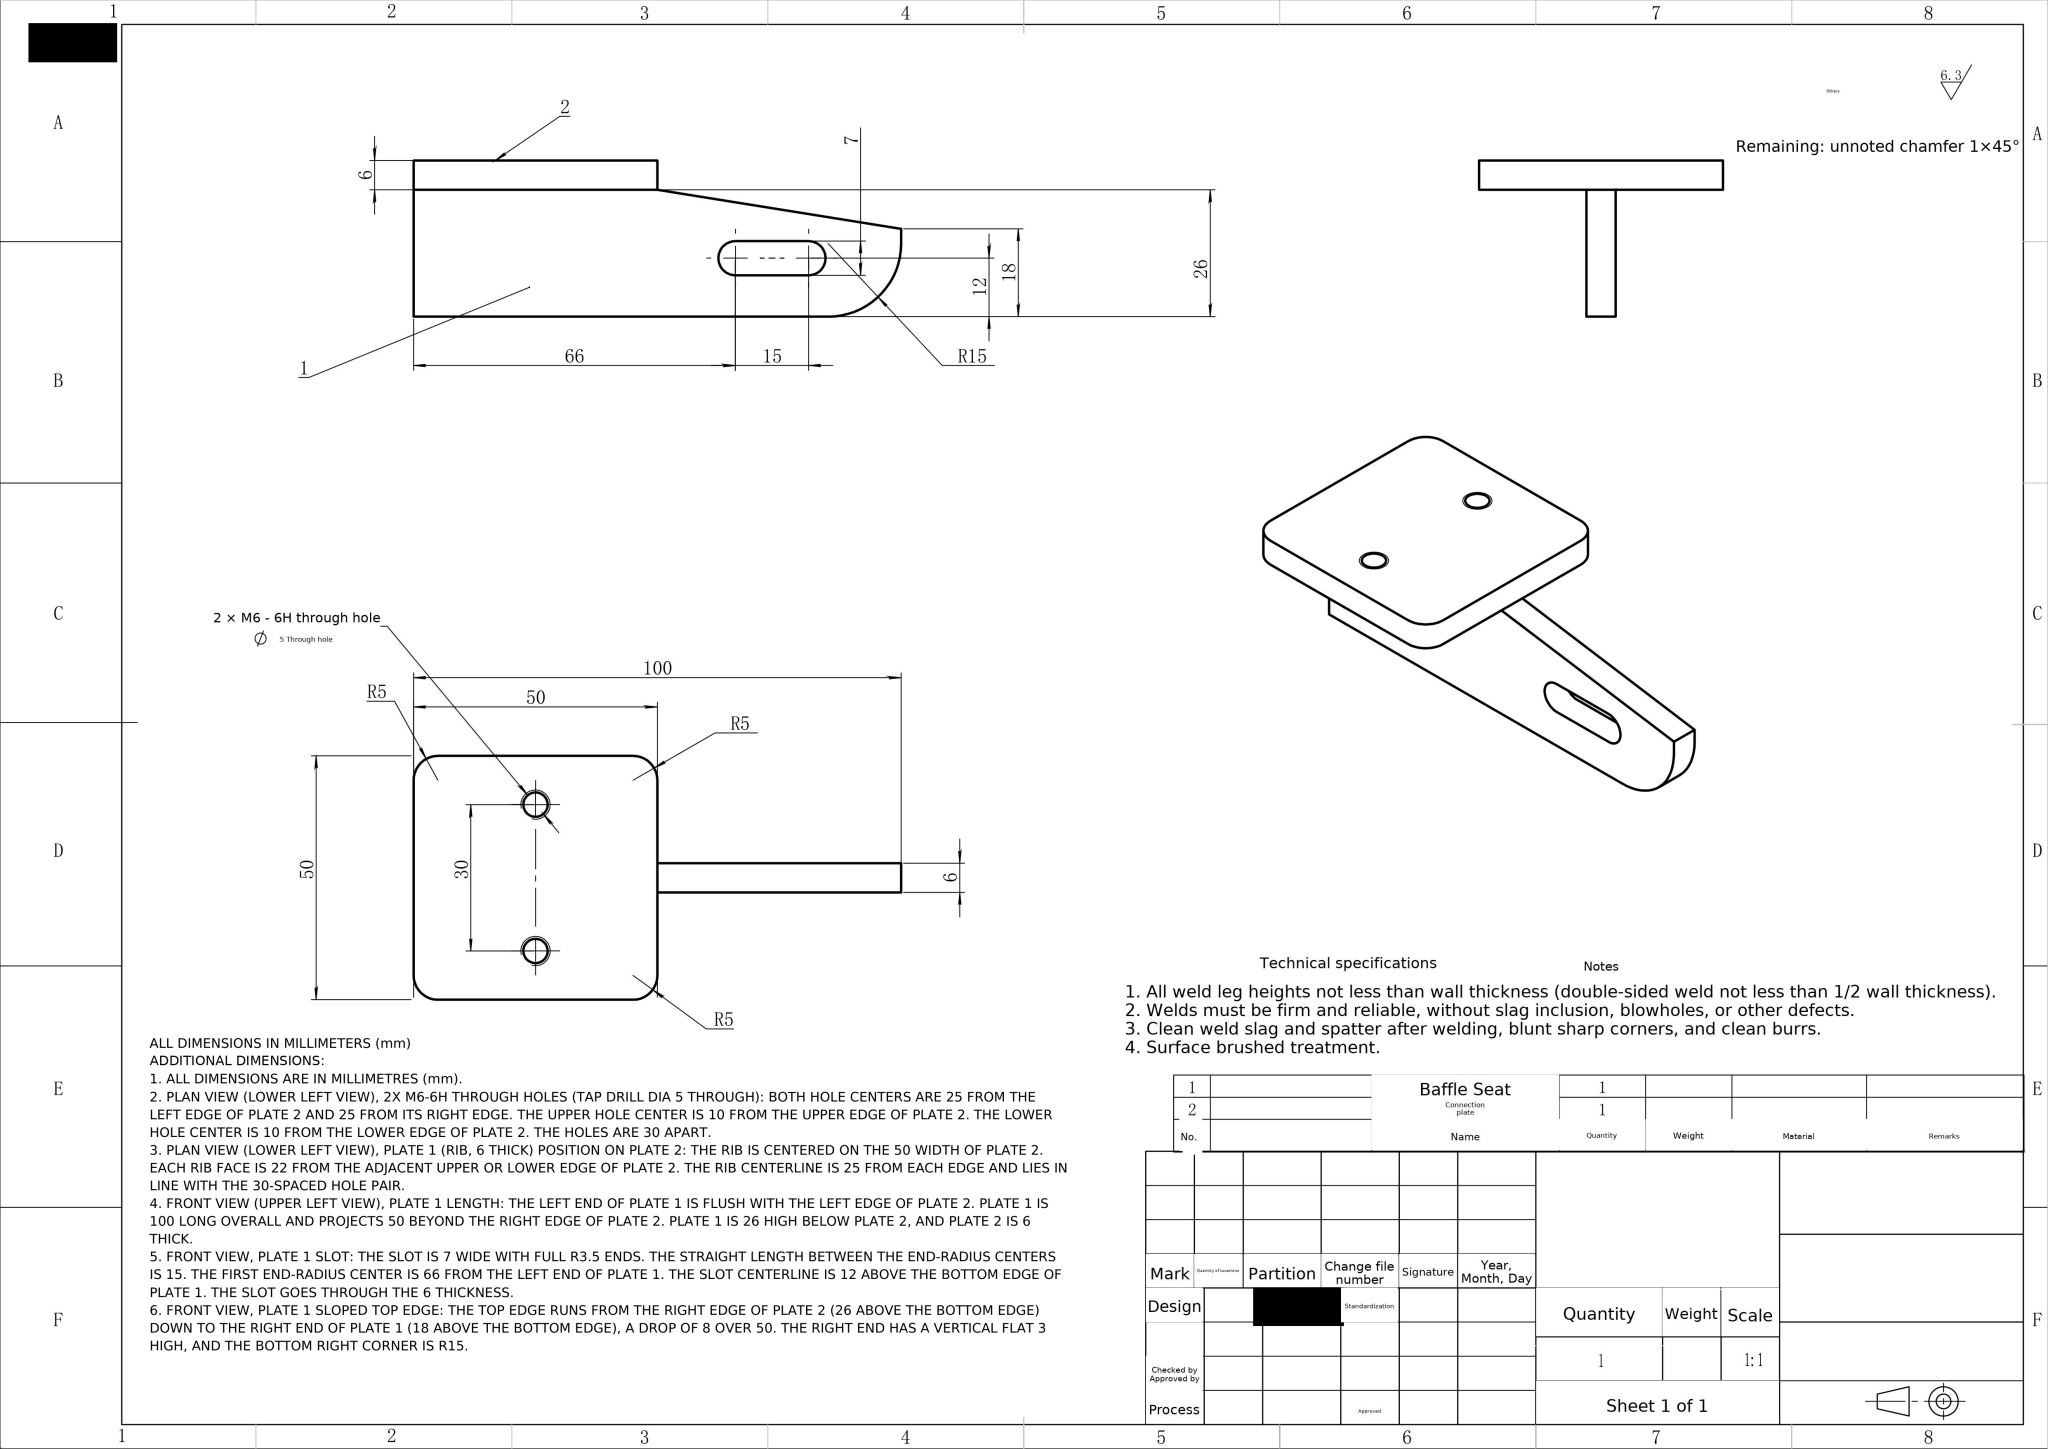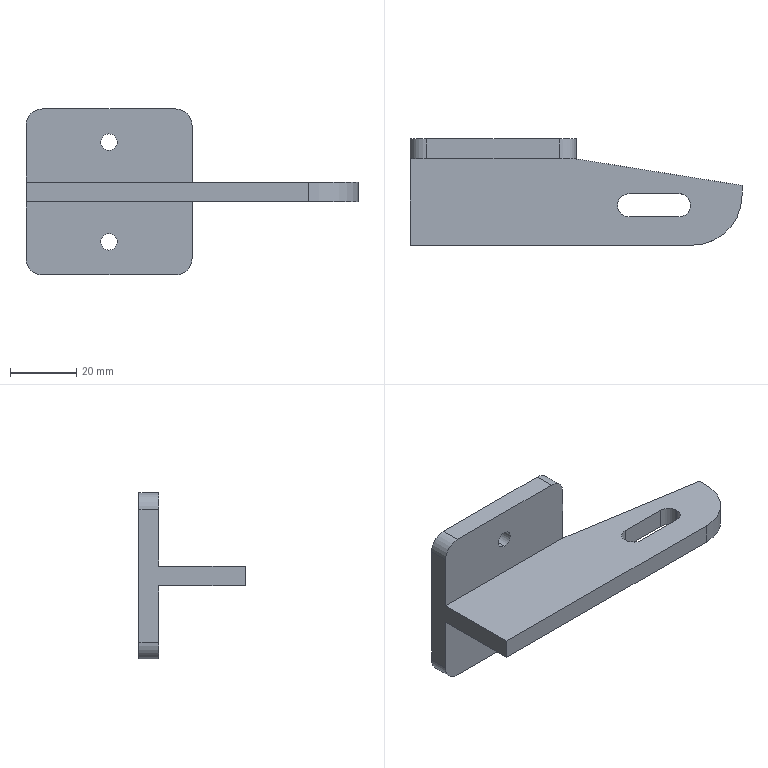Part | NX | mm | L-Shaped Slotted Foot Plate | 1 solid | 26 faces | box 100 x 32 x 50 mm | volume 27885 mm3 | plane 14 | cylinder 12 | commonest cylinder face diameters 5 x4 10 x4 7 x3 30 x1
STEP:
#1=COLOUR_RGB('',0.7922,0.8196,0.9333);
#2=FILL_AREA_STYLE_COLOUR('',#1);
#3=FILL_AREA_STYLE('',(#2));
#4=SURFACE_STYLE_FILL_AREA(#3);
#5=SURFACE_SIDE_STYLE('',(#4));
#6=SURFACE_STYLE_USAGE(.BOTH.,#5);
#7=PRESENTATION_STYLE_ASSIGNMENT((#6));
#8=CARTESIAN_POINT('',(31.,-17.5,-28.));
#9=VERTEX_POINT('',#8);
#10=CARTESIAN_POINT('',(16.,-17.5,-28.));
#11=VERTEX_POINT('',#10);
#12=CARTESIAN_POINT('',(16.,-17.5,-28.));
#13=DIRECTION('',(-1.,-0.,0.));
#14=VECTOR('',#13,1000.);
#15=LINE('',#12,#14);
#16=EDGE_CURVE('',#9,#11,#15,.T.);
#17=ORIENTED_EDGE('',*,*,#16,.T.);
#18=CARTESIAN_POINT('',(16.,-17.5,-22.));
#19=VERTEX_POINT('',#18);
#20=CARTESIAN_POINT('',(16.,-17.5,-50.001));
#21=DIRECTION('',(-0.,0.,1.));
#22=VECTOR('',#21,1000.);
#23=LINE('',#20,#22);
#24=EDGE_CURVE('',#11,#19,#23,.T.);
#25=ORIENTED_EDGE('',*,*,#24,.T.);
#26=CARTESIAN_POINT('',(31.,-17.5,-22.));
#27=VERTEX_POINT('',#26);
#28=CARTESIAN_POINT('',(16.,-17.5,-22.));
#29=DIRECTION('',(1.,0.,-0.));
#30=VECTOR('',#29,1000.);
#31=LINE('',#28,#30);
#32=EDGE_CURVE('',#19,#27,#31,.T.);
#33=ORIENTED_EDGE('',*,*,#32,.T.);
#34=CARTESIAN_POINT('',(31.,-17.5,-50.001));
#35=DIRECTION('',(-0.,0.,1.));
#36=VECTOR('',#35,1000.);
#37=LINE('',#34,#36);
#38=EDGE_CURVE('',#9,#27,#37,.T.);
#39=ORIENTED_EDGE('',*,*,#38,.F.);
#40=EDGE_LOOP('',(#17,#25,#33,#39));
#41=FACE_OUTER_BOUND('',#40,.T.);
#42=CARTESIAN_POINT('',(16.,-17.5,-50.001));
#43=DIRECTION('',(-0.,-1.,0.));
#44=DIRECTION('',(-1.,0.,0.));
#45=AXIS2_PLACEMENT_3D('',#42,#43,#44);
#46=PLANE('',#45);
#47=ADVANCED_FACE('',(#41),#46,.F.);
#48=CARTESIAN_POINT('',(34.5,-14.,-28.));
#49=VERTEX_POINT('',#48);
#50=CARTESIAN_POINT('',(34.5,-14.,-22.));
#51=VERTEX_POINT('',#50);
#52=CARTESIAN_POINT('',(34.5,-14.,-50.001));
#53=DIRECTION('',(-0.,0.,1.));
#54=VECTOR('',#53,1000.);
#55=LINE('',#52,#54);
#56=EDGE_CURVE('',#49,#51,#55,.T.);
#57=ORIENTED_EDGE('',*,*,#56,.F.);
#58=CARTESIAN_POINT('',(31.,-14.,-28.));
#59=DIRECTION('',(0.,-0.,-1.));
#60=DIRECTION('',(1.,0.,0.));
#61=AXIS2_PLACEMENT_3D('',#58,#59,#60);
#62=CIRCLE('',#61,3.5);
#63=EDGE_CURVE('',#49,#9,#62,.T.);
#64=ORIENTED_EDGE('',*,*,#63,.T.);
#65=ORIENTED_EDGE('',*,*,#38,.T.);
#66=CARTESIAN_POINT('',(31.,-14.,-22.));
#67=DIRECTION('',(-0.,0.,1.));
#68=DIRECTION('',(1.,0.,0.));
#69=AXIS2_PLACEMENT_3D('',#66,#67,#68);
#70=CIRCLE('',#69,3.5);
#71=EDGE_CURVE('',#27,#51,#70,.T.);
#72=ORIENTED_EDGE('',*,*,#71,.T.);
#73=EDGE_LOOP('',(#57,#64,#65,#72));
#74=FACE_OUTER_BOUND('',#73,.T.);
#75=CARTESIAN_POINT('',(31.,-14.,-50.001));
#76=DIRECTION('',(-0.,0.,1.));
#77=DIRECTION('',(1.,0.,0.));
#78=AXIS2_PLACEMENT_3D('',#75,#76,#77);
#79=CYLINDRICAL_SURFACE('',#78,3.5);
#80=ADVANCED_FACE('',(#74),#79,.F.);
#81=CARTESIAN_POINT('',(16.,-10.5,-28.));
#82=VERTEX_POINT('',#81);
#83=CARTESIAN_POINT('',(31.,-10.5,-28.));
#84=VERTEX_POINT('',#83);
#85=CARTESIAN_POINT('',(16.,-10.5,-28.));
#86=DIRECTION('',(1.,0.,-0.));
#87=VECTOR('',#86,1000.);
#88=LINE('',#85,#87);
#89=EDGE_CURVE('',#82,#84,#88,.T.);
#90=ORIENTED_EDGE('',*,*,#89,.T.);
#91=CARTESIAN_POINT('',(31.,-10.5,-22.));
#92=VERTEX_POINT('',#91);
#93=CARTESIAN_POINT('',(31.,-10.5,-50.001));
#94=DIRECTION('',(-0.,0.,1.));
#95=VECTOR('',#94,1000.);
#96=LINE('',#93,#95);
#97=EDGE_CURVE('',#84,#92,#96,.T.);
#98=ORIENTED_EDGE('',*,*,#97,.T.);
#99=CARTESIAN_POINT('',(16.,-10.5,-22.));
#100=VERTEX_POINT('',#99);
#101=CARTESIAN_POINT('',(16.,-10.5,-22.));
#102=DIRECTION('',(-1.,-0.,0.));
#103=VECTOR('',#102,1000.);
#104=LINE('',#101,#103);
#105=EDGE_CURVE('',#92,#100,#104,.T.);
#106=ORIENTED_EDGE('',*,*,#105,.T.);
#107=CARTESIAN_POINT('',(16.,-10.5,-50.001));
#108=DIRECTION('',(-0.,0.,1.));
#109=VECTOR('',#108,1000.);
#110=LINE('',#107,#109);
#111=EDGE_CURVE('',#82,#100,#110,.T.);
#112=ORIENTED_EDGE('',*,*,#111,.F.);
#113=EDGE_LOOP('',(#90,#98,#106,#112));
#114=FACE_OUTER_BOUND('',#113,.T.);
#115=CARTESIAN_POINT('',(16.,-10.5,-50.001));
#116=DIRECTION('',(0.,1.,-0.));
#117=DIRECTION('',(1.,-0.,0.));
#118=AXIS2_PLACEMENT_3D('',#115,#116,#117);
#119=PLANE('',#118);
#120=ADVANCED_FACE('',(#114),#119,.F.);
#121=CARTESIAN_POINT('',(16.,-14.,-28.));
#122=DIRECTION('',(0.,-0.,-1.));
#123=DIRECTION('',(1.,0.,0.));
#124=AXIS2_PLACEMENT_3D('',#121,#122,#123);
#125=CIRCLE('',#124,3.5);
#126=EDGE_CURVE('',#11,#82,#125,.T.);
#127=ORIENTED_EDGE('',*,*,#126,.T.);
#128=ORIENTED_EDGE('',*,*,#111,.T.);
#129=CARTESIAN_POINT('',(16.,-14.,-22.));
#130=DIRECTION('',(-0.,0.,1.));
#131=DIRECTION('',(1.,0.,0.));
#132=AXIS2_PLACEMENT_3D('',#129,#130,#131);
#133=CIRCLE('',#132,3.5);
#134=EDGE_CURVE('',#100,#19,#133,.T.);
#135=ORIENTED_EDGE('',*,*,#134,.T.);
#136=ORIENTED_EDGE('',*,*,#24,.F.);
#137=EDGE_LOOP('',(#127,#128,#135,#136));
#138=FACE_OUTER_BOUND('',#137,.T.);
#139=CARTESIAN_POINT('',(16.,-14.,-50.001));
#140=DIRECTION('',(-0.,0.,1.));
#141=DIRECTION('',(1.,0.,0.));
#142=AXIS2_PLACEMENT_3D('',#139,#140,#141);
#143=CYLINDRICAL_SURFACE('',#142,3.5);
#144=ADVANCED_FACE('',(#138),#143,.F.);
#145=CARTESIAN_POINT('',(50.,-11.,-28.));
#146=VERTEX_POINT('',#145);
#147=CARTESIAN_POINT('',(35.,-26.,-28.));
#148=VERTEX_POINT('',#147);
#149=CARTESIAN_POINT('',(35.,-11.,-28.));
#150=DIRECTION('',(-0.,-0.,-1.));
#151=DIRECTION('',(1.,-0.,0.));
#152=AXIS2_PLACEMENT_3D('',#149,#150,#151);
#153=CIRCLE('',#152,15.);
#154=EDGE_CURVE('',#146,#148,#153,.T.);
#155=ORIENTED_EDGE('',*,*,#154,.F.);
#156=CARTESIAN_POINT('',(50.,-11.,-22.));
#157=VERTEX_POINT('',#156);
#158=CARTESIAN_POINT('',(50.,-11.,-28.));
#159=DIRECTION('',(0.,-0.,-1.));
#160=VECTOR('',#159,1000.);
#161=LINE('',#158,#160);
#162=EDGE_CURVE('',#157,#146,#161,.T.);
#163=ORIENTED_EDGE('',*,*,#162,.F.);
#164=CARTESIAN_POINT('',(35.,-26.,-22.));
#165=VERTEX_POINT('',#164);
#166=CARTESIAN_POINT('',(35.,-11.,-22.));
#167=DIRECTION('',(-0.,0.,1.));
#168=DIRECTION('',(-1.,-0.,-0.));
#169=AXIS2_PLACEMENT_3D('',#166,#167,#168);
#170=CIRCLE('',#169,15.);
#171=EDGE_CURVE('',#165,#157,#170,.T.);
#172=ORIENTED_EDGE('',*,*,#171,.F.);
#173=CARTESIAN_POINT('',(35.,-26.,-22.));
#174=DIRECTION('',(-0.,0.,1.));
#175=VECTOR('',#174,1000.);
#176=LINE('',#173,#175);
#177=EDGE_CURVE('',#148,#165,#176,.T.);
#178=ORIENTED_EDGE('',*,*,#177,.F.);
#179=EDGE_LOOP('',(#155,#163,#172,#178));
#180=FACE_OUTER_BOUND('',#179,.T.);
#181=CARTESIAN_POINT('',(35.,-11.,-28.));
#182=DIRECTION('',(0.,-0.,-1.));
#183=DIRECTION('',(-1.,-0.,-0.));
#184=AXIS2_PLACEMENT_3D('',#181,#182,#183);
#185=CYLINDRICAL_SURFACE('',#184,15.);
#186=ADVANCED_FACE('',(#180),#185,.T.);
#187=CARTESIAN_POINT('',(50.,-8.,-22.));
#188=VERTEX_POINT('',#187);
#189=CARTESIAN_POINT('',(50.,-8.,-28.));
#190=VERTEX_POINT('',#189);
#191=CARTESIAN_POINT('',(50.,-8.,158.366));
#192=DIRECTION('',(0.,-0.,-1.));
#193=VECTOR('',#192,1000.);
#194=LINE('',#191,#193);
#195=EDGE_CURVE('',#188,#190,#194,.T.);
#196=ORIENTED_EDGE('',*,*,#195,.T.);
#197=CARTESIAN_POINT('',(0.,-0.,-28.));
#198=VERTEX_POINT('',#197);
#199=CARTESIAN_POINT('',(-44.696,7.151,-28.));
#200=DIRECTION('',(-0.9874,0.158,0.));
#201=VECTOR('',#200,1000.);
#202=LINE('',#199,#201);
#203=EDGE_CURVE('',#190,#198,#202,.T.);
#204=ORIENTED_EDGE('',*,*,#203,.T.);
#205=CARTESIAN_POINT('',(0.,-0.,-22.));
#206=VERTEX_POINT('',#205);
#207=CARTESIAN_POINT('',(0.,0.,-28.));
#208=DIRECTION('',(-0.,0.,1.));
#209=VECTOR('',#208,1000.);
#210=LINE('',#207,#209);
#211=EDGE_CURVE('',#198,#206,#210,.T.);
#212=ORIENTED_EDGE('',*,*,#211,.T.);
#213=CARTESIAN_POINT('',(-44.696,7.151,-22.));
#214=DIRECTION('',(0.9874,-0.158,0.));
#215=VECTOR('',#214,1000.);
#216=LINE('',#213,#215);
#217=EDGE_CURVE('',#206,#188,#216,.T.);
#218=ORIENTED_EDGE('',*,*,#217,.T.);
#219=EDGE_LOOP('',(#196,#204,#212,#218));
#220=FACE_OUTER_BOUND('',#219,.T.);
#221=CARTESIAN_POINT('',(0.,0.,158.366));
#222=DIRECTION('',(0.158,0.9874,0.));
#223=DIRECTION('',(0.,0.,-1.));
#224=AXIS2_PLACEMENT_3D('',#221,#222,#223);
#225=PLANE('',#224);
#226=ADVANCED_FACE('',(#220),#225,.T.);
#227=CARTESIAN_POINT('',(-50.,-26.,-28.));
#228=VERTEX_POINT('',#227);
#229=CARTESIAN_POINT('',(-50.,-26.,-28.));
#230=DIRECTION('',(1.,0.,-0.));
#231=VECTOR('',#230,1000.);
#232=LINE('',#229,#231);
#233=EDGE_CURVE('',#228,#148,#232,.T.);
#234=ORIENTED_EDGE('',*,*,#233,.T.);
#235=ORIENTED_EDGE('',*,*,#177,.T.);
#236=CARTESIAN_POINT('',(-50.,-26.,-22.));
#237=VERTEX_POINT('',#236);
#238=CARTESIAN_POINT('',(-50.,-26.,-22.));
#239=DIRECTION('',(-1.,-0.,-0.));
#240=VECTOR('',#239,1000.);
#241=LINE('',#238,#240);
#242=EDGE_CURVE('',#165,#237,#241,.T.);
#243=ORIENTED_EDGE('',*,*,#242,.T.);
#244=CARTESIAN_POINT('',(-50.,-26.,-22.));
#245=DIRECTION('',(0.,-0.,-1.));
#246=VECTOR('',#245,1000.);
#247=LINE('',#244,#246);
#248=EDGE_CURVE('',#237,#228,#247,.T.);
#249=ORIENTED_EDGE('',*,*,#248,.T.);
#250=EDGE_LOOP('',(#234,#235,#243,#249));
#251=FACE_OUTER_BOUND('',#250,.T.);
#252=CARTESIAN_POINT('',(-50.,-26.,-28.));
#253=DIRECTION('',(-0.,-1.,0.));
#254=DIRECTION('',(-1.,0.,0.));
#255=AXIS2_PLACEMENT_3D('',#252,#253,#254);
#256=PLANE('',#255);
#257=ADVANCED_FACE('',(#251),#256,.T.);
#258=CARTESIAN_POINT('',(-50.,-0.,-22.));
#259=VERTEX_POINT('',#258);
#260=CARTESIAN_POINT('',(-50.,-26.,-22.));
#261=DIRECTION('',(0.,1.,0.));
#262=VECTOR('',#261,1000.);
#263=LINE('',#260,#262);
#264=EDGE_CURVE('',#237,#259,#263,.T.);
#265=ORIENTED_EDGE('',*,*,#264,.T.);
#266=CARTESIAN_POINT('',(-50.,-0.,-5.));
#267=VERTEX_POINT('',#266);
#268=CARTESIAN_POINT('',(-50.,-0.,-5.));
#269=DIRECTION('',(-0.,0.,1.));
#270=VECTOR('',#269,1000.);
#271=LINE('',#268,#270);
#272=EDGE_CURVE('',#259,#267,#271,.T.);
#273=ORIENTED_EDGE('',*,*,#272,.T.);
#274=CARTESIAN_POINT('',(-50.,6.,-5.));
#275=VERTEX_POINT('',#274);
#276=CARTESIAN_POINT('',(-50.,6.,-5.));
#277=DIRECTION('',(-0.,-1.,-0.));
#278=VECTOR('',#277,1000.);
#279=LINE('',#276,#278);
#280=EDGE_CURVE('',#275,#267,#279,.T.);
#281=ORIENTED_EDGE('',*,*,#280,.F.);
#282=CARTESIAN_POINT('',(-50.,6.,-45.));
#283=VERTEX_POINT('',#282);
#284=CARTESIAN_POINT('',(-50.,6.,-5.));
#285=DIRECTION('',(-0.,0.,1.));
#286=VECTOR('',#285,1000.);
#287=LINE('',#284,#286);
#288=EDGE_CURVE('',#283,#275,#287,.T.);
#289=ORIENTED_EDGE('',*,*,#288,.F.);
#290=CARTESIAN_POINT('',(-50.,-0.,-45.));
#291=VERTEX_POINT('',#290);
#292=CARTESIAN_POINT('',(-50.,6.,-45.));
#293=DIRECTION('',(-0.,-1.,-0.));
#294=VECTOR('',#293,1000.);
#295=LINE('',#292,#294);
#296=EDGE_CURVE('',#283,#291,#295,.T.);
#297=ORIENTED_EDGE('',*,*,#296,.T.);
#298=CARTESIAN_POINT('',(-50.,-0.,-28.));
#299=VERTEX_POINT('',#298);
#300=CARTESIAN_POINT('',(-50.,-0.,-5.));
#301=DIRECTION('',(-0.,0.,1.));
#302=VECTOR('',#301,1000.);
#303=LINE('',#300,#302);
#304=EDGE_CURVE('',#291,#299,#303,.T.);
#305=ORIENTED_EDGE('',*,*,#304,.T.);
#306=CARTESIAN_POINT('',(-50.,-26.,-28.));
#307=DIRECTION('',(0.,1.,0.));
#308=VECTOR('',#307,1000.);
#309=LINE('',#306,#308);
#310=EDGE_CURVE('',#228,#299,#309,.T.);
#311=ORIENTED_EDGE('',*,*,#310,.F.);
#312=ORIENTED_EDGE('',*,*,#248,.F.);
#313=EDGE_LOOP('',(#265,#273,#281,#289,#297,#305,#311,#312));
#314=FACE_OUTER_BOUND('',#313,.T.);
#315=CARTESIAN_POINT('',(-50.,-26.,-22.));
#316=DIRECTION('',(1.,0.,0.));
#317=DIRECTION('',(-0.,1.,0.));
#318=AXIS2_PLACEMENT_3D('',#315,#316,#317);
#319=PLANE('',#318);
#320=ADVANCED_FACE('',(#314),#319,.F.);
#321=ORIENTED_EDGE('',*,*,#32,.F.);
#322=ORIENTED_EDGE('',*,*,#134,.F.);
#323=ORIENTED_EDGE('',*,*,#105,.F.);
#324=CARTESIAN_POINT('',(31.,-14.,-22.));
#325=DIRECTION('',(-0.,0.,1.));
#326=DIRECTION('',(1.,0.,0.));
#327=AXIS2_PLACEMENT_3D('',#324,#325,#326);
#328=CIRCLE('',#327,3.5);
#329=EDGE_CURVE('',#51,#92,#328,.T.);
#330=ORIENTED_EDGE('',*,*,#329,.F.);
#331=ORIENTED_EDGE('',*,*,#71,.F.);
#332=EDGE_LOOP('',(#321,#322,#323,#330,#331));
#333=FACE_BOUND('',#332,.T.);
#334=ORIENTED_EDGE('',*,*,#242,.F.);
#335=ORIENTED_EDGE('',*,*,#171,.T.);
#336=CARTESIAN_POINT('',(50.,-26.,-22.));
#337=DIRECTION('',(0.,1.,0.));
#338=VECTOR('',#337,1000.);
#339=LINE('',#336,#338);
#340=EDGE_CURVE('',#157,#188,#339,.T.);
#341=ORIENTED_EDGE('',*,*,#340,.T.);
#342=ORIENTED_EDGE('',*,*,#217,.F.);
#343=CARTESIAN_POINT('',(-50.,-0.,-22.));
#344=DIRECTION('',(-1.,-0.,-0.));
#345=VECTOR('',#344,1000.);
#346=LINE('',#343,#345);
#347=EDGE_CURVE('',#206,#259,#346,.T.);
#348=ORIENTED_EDGE('',*,*,#347,.T.);
#349=ORIENTED_EDGE('',*,*,#264,.F.);
#350=EDGE_LOOP('',(#334,#335,#341,#342,#348,#349));
#351=FACE_OUTER_BOUND('',#350,.T.);
#352=CARTESIAN_POINT('',(-50.,-26.,-22.));
#353=DIRECTION('',(0.,-0.,-1.));
#354=DIRECTION('',(0.,-1.,0.));
#355=AXIS2_PLACEMENT_3D('',#352,#353,#354);
#356=PLANE('',#355);
#357=ADVANCED_FACE('',(#333,#351),#356,.F.);
#358=ORIENTED_EDGE('',*,*,#340,.F.);
#359=ORIENTED_EDGE('',*,*,#162,.T.);
#360=CARTESIAN_POINT('',(50.,-26.,-28.));
#361=DIRECTION('',(0.,1.,0.));
#362=VECTOR('',#361,1000.);
#363=LINE('',#360,#362);
#364=EDGE_CURVE('',#146,#190,#363,.T.);
#365=ORIENTED_EDGE('',*,*,#364,.T.);
#366=ORIENTED_EDGE('',*,*,#195,.F.);
#367=EDGE_LOOP('',(#358,#359,#365,#366));
#368=FACE_OUTER_BOUND('',#367,.T.);
#369=CARTESIAN_POINT('',(50.,-26.,-22.));
#370=DIRECTION('',(-1.,-0.,-0.));
#371=DIRECTION('',(-0.,0.,1.));
#372=AXIS2_PLACEMENT_3D('',#369,#370,#371);
#373=PLANE('',#372);
#374=ADVANCED_FACE('',(#368),#373,.F.);
#375=ORIENTED_EDGE('',*,*,#89,.F.);
#376=ORIENTED_EDGE('',*,*,#126,.F.);
#377=ORIENTED_EDGE('',*,*,#16,.F.);
#378=ORIENTED_EDGE('',*,*,#63,.F.);
#379=CARTESIAN_POINT('',(31.,-14.,-28.));
#380=DIRECTION('',(-0.,-0.,-1.));
#381=DIRECTION('',(1.,-0.,0.));
#382=AXIS2_PLACEMENT_3D('',#379,#380,#381);
#383=CIRCLE('',#382,3.5);
#384=EDGE_CURVE('',#84,#49,#383,.T.);
#385=ORIENTED_EDGE('',*,*,#384,.F.);
#386=EDGE_LOOP('',(#375,#376,#377,#378,#385));
#387=FACE_BOUND('',#386,.T.);
#388=ORIENTED_EDGE('',*,*,#364,.F.);
#389=ORIENTED_EDGE('',*,*,#154,.T.);
#390=ORIENTED_EDGE('',*,*,#233,.F.);
#391=ORIENTED_EDGE('',*,*,#310,.T.);
#392=CARTESIAN_POINT('',(-50.,-0.,-28.));
#393=DIRECTION('',(1.,0.,-0.));
#394=VECTOR('',#393,1000.);
#395=LINE('',#392,#394);
#396=EDGE_CURVE('',#299,#198,#395,.T.);
#397=ORIENTED_EDGE('',*,*,#396,.T.);
#398=ORIENTED_EDGE('',*,*,#203,.F.);
#399=EDGE_LOOP('',(#388,#389,#390,#391,#397,#398));
#400=FACE_OUTER_BOUND('',#399,.T.);
#401=CARTESIAN_POINT('',(-50.,-26.,-28.));
#402=DIRECTION('',(0.,0.,1.));
#403=DIRECTION('',(0.,-1.,0.));
#404=AXIS2_PLACEMENT_3D('',#401,#402,#403);
#405=PLANE('',#404);
#406=ADVANCED_FACE('',(#387,#400),#405,.F.);
#407=ORIENTED_EDGE('',*,*,#384,.T.);
#408=ORIENTED_EDGE('',*,*,#56,.T.);
#409=ORIENTED_EDGE('',*,*,#329,.T.);
#410=ORIENTED_EDGE('',*,*,#97,.F.);
#411=EDGE_LOOP('',(#407,#408,#409,#410));
#412=FACE_OUTER_BOUND('',#411,.T.);
#413=CARTESIAN_POINT('',(31.,-14.,-50.001));
#414=DIRECTION('',(-0.,0.,1.));
#415=DIRECTION('',(1.,0.,0.));
#416=AXIS2_PLACEMENT_3D('',#413,#414,#415);
#417=CYLINDRICAL_SURFACE('',#416,3.5);
#418=ADVANCED_FACE('',(#412),#417,.F.);
#419=CARTESIAN_POINT('',(-25.,-0.,-37.5));
#420=VERTEX_POINT('',#419);
#421=CARTESIAN_POINT('',(-25.,0.,-42.5));
#422=VERTEX_POINT('',#421);
#423=CARTESIAN_POINT('',(-25.,0.,-40.));
#424=DIRECTION('',(-0.,-1.,0.));
#425=DIRECTION('',(0.,-0.,-1.));
#426=AXIS2_PLACEMENT_3D('',#423,#424,#425);
#427=CIRCLE('',#426,2.5);
#428=EDGE_CURVE('',#420,#422,#427,.T.);
#429=ORIENTED_EDGE('',*,*,#428,.F.);
#430=CARTESIAN_POINT('',(-25.,0.,-40.));
#431=DIRECTION('',(-0.,-1.,0.));
#432=DIRECTION('',(0.,-0.,-1.));
#433=AXIS2_PLACEMENT_3D('',#430,#431,#432);
#434=CIRCLE('',#433,2.5);
#435=EDGE_CURVE('',#422,#420,#434,.T.);
#436=ORIENTED_EDGE('',*,*,#435,.F.);
#437=EDGE_LOOP('',(#429,#436));
#438=FACE_BOUND('',#437,.T.);
#439=ORIENTED_EDGE('',*,*,#396,.F.);
#440=ORIENTED_EDGE('',*,*,#304,.F.);
#441=CARTESIAN_POINT('',(-45.,-0.,-50.));
#442=VERTEX_POINT('',#441);
#443=CARTESIAN_POINT('',(-45.,-0.,-45.));
#444=DIRECTION('',(0.,1.,-0.));
#445=DIRECTION('',(0.,0.,1.));
#446=AXIS2_PLACEMENT_3D('',#443,#444,#445);
#447=CIRCLE('',#446,5.);
#448=EDGE_CURVE('',#442,#291,#447,.T.);
#449=ORIENTED_EDGE('',*,*,#448,.F.);
#450=CARTESIAN_POINT('',(-5.,0.,-50.));
#451=VERTEX_POINT('',#450);
#452=CARTESIAN_POINT('',(-5.,0.,-50.));
#453=DIRECTION('',(-1.,-0.,0.));
#454=VECTOR('',#453,1000.);
#455=LINE('',#452,#454);
#456=EDGE_CURVE('',#451,#442,#455,.T.);
#457=ORIENTED_EDGE('',*,*,#456,.F.);
#458=CARTESIAN_POINT('',(0.,0.,-45.));
#459=VERTEX_POINT('',#458);
#460=CARTESIAN_POINT('',(-5.,0.,-45.));
#461=DIRECTION('',(0.,1.,-0.));
#462=DIRECTION('',(0.,-0.,-1.));
#463=AXIS2_PLACEMENT_3D('',#460,#461,#462);
#464=CIRCLE('',#463,5.);
#465=EDGE_CURVE('',#459,#451,#464,.T.);
#466=ORIENTED_EDGE('',*,*,#465,.F.);
#467=CARTESIAN_POINT('',(0.,0.,-5.));
#468=DIRECTION('',(0.,-0.,-1.));
#469=VECTOR('',#468,1000.);
#470=LINE('',#467,#469);
#471=EDGE_CURVE('',#198,#459,#470,.T.);
#472=ORIENTED_EDGE('',*,*,#471,.F.);
#473=EDGE_LOOP('',(#439,#440,#449,#457,#466,#472));
#474=FACE_OUTER_BOUND('',#473,.T.);
#475=CARTESIAN_POINT('',(-5.,0.,-45.));
#476=DIRECTION('',(-0.,-1.,0.));
#477=DIRECTION('',(-1.,0.,0.));
#478=AXIS2_PLACEMENT_3D('',#475,#476,#477);
#479=PLANE('',#478);
#480=ADVANCED_FACE('',(#438,#474),#479,.T.);
#481=CARTESIAN_POINT('',(-25.,-0.,-7.5));
#482=VERTEX_POINT('',#481);
#483=CARTESIAN_POINT('',(-25.,0.,-12.5));
#484=VERTEX_POINT('',#483);
#485=CARTESIAN_POINT('',(-25.,0.,-10.));
#486=DIRECTION('',(-0.,-1.,0.));
#487=DIRECTION('',(0.,-0.,-1.));
#488=AXIS2_PLACEMENT_3D('',#485,#486,#487);
#489=CIRCLE('',#488,2.5);
#490=EDGE_CURVE('',#482,#484,#489,.T.);
#491=ORIENTED_EDGE('',*,*,#490,.F.);
#492=CARTESIAN_POINT('',(-25.,0.,-10.));
#493=DIRECTION('',(-0.,-1.,0.));
#494=DIRECTION('',(0.,-0.,-1.));
#495=AXIS2_PLACEMENT_3D('',#492,#493,#494);
#496=CIRCLE('',#495,2.5);
#497=EDGE_CURVE('',#484,#482,#496,.T.);
#498=ORIENTED_EDGE('',*,*,#497,.F.);
#499=EDGE_LOOP('',(#491,#498));
#500=FACE_BOUND('',#499,.T.);
#501=ORIENTED_EDGE('',*,*,#347,.F.);
#502=CARTESIAN_POINT('',(0.,0.,-5.));
#503=VERTEX_POINT('',#502);
#504=CARTESIAN_POINT('',(0.,0.,-5.));
#505=DIRECTION('',(0.,-0.,-1.));
#506=VECTOR('',#505,1000.);
#507=LINE('',#504,#506);
#508=EDGE_CURVE('',#503,#206,#507,.T.);
#509=ORIENTED_EDGE('',*,*,#508,.F.);
#510=CARTESIAN_POINT('',(-5.,0.,0.));
#511=VERTEX_POINT('',#510);
#512=CARTESIAN_POINT('',(-5.,0.,-5.));
#513=DIRECTION('',(0.,1.,-0.));
#514=DIRECTION('',(0.,-0.,-1.));
#515=AXIS2_PLACEMENT_3D('',#512,#513,#514);
#516=CIRCLE('',#515,5.);
#517=EDGE_CURVE('',#511,#503,#516,.T.);
#518=ORIENTED_EDGE('',*,*,#517,.F.);
#519=CARTESIAN_POINT('',(-45.,-0.,0.));
#520=VERTEX_POINT('',#519);
#521=CARTESIAN_POINT('',(-5.,0.,0.));
#522=DIRECTION('',(1.,0.,-0.));
#523=VECTOR('',#522,1000.);
#524=LINE('',#521,#523);
#525=EDGE_CURVE('',#520,#511,#524,.T.);
#526=ORIENTED_EDGE('',*,*,#525,.F.);
#527=CARTESIAN_POINT('',(-45.,-0.,-5.));
#528=DIRECTION('',(0.,1.,-0.));
#529=DIRECTION('',(0.,-0.,-1.));
#530=AXIS2_PLACEMENT_3D('',#527,#528,#529);
#531=CIRCLE('',#530,5.);
#532=EDGE_CURVE('',#267,#520,#531,.T.);
#533=ORIENTED_EDGE('',*,*,#532,.F.);
#534=ORIENTED_EDGE('',*,*,#272,.F.);
#535=EDGE_LOOP('',(#501,#509,#518,#526,#533,#534));
#536=FACE_OUTER_BOUND('',#535,.T.);
#537=CARTESIAN_POINT('',(-5.,0.,-45.));
#538=DIRECTION('',(-0.,-1.,0.));
#539=DIRECTION('',(-1.,0.,0.));
#540=AXIS2_PLACEMENT_3D('',#537,#538,#539);
#541=PLANE('',#540);
#542=ADVANCED_FACE('',(#500,#536),#541,.T.);
#543=CARTESIAN_POINT('',(-25.,6.,-42.5));
#544=VERTEX_POINT('',#543);
#545=CARTESIAN_POINT('',(-25.,6.,-42.5));
#546=DIRECTION('',(0.,1.,0.));
#547=VECTOR('',#546,1000.);
#548=LINE('',#545,#547);
#549=EDGE_CURVE('',#422,#544,#548,.T.);
#550=ORIENTED_EDGE('',*,*,#549,.F.);
#551=ORIENTED_EDGE('',*,*,#435,.T.);
#552=CARTESIAN_POINT('',(-25.,6.,-37.5));
#553=VERTEX_POINT('',#552);
#554=CARTESIAN_POINT('',(-25.,6.,-37.5));
#555=DIRECTION('',(0.,1.,0.));
#556=VECTOR('',#555,1000.);
#557=LINE('',#554,#556);
#558=EDGE_CURVE('',#420,#553,#557,.T.);
#559=ORIENTED_EDGE('',*,*,#558,.T.);
#560=CARTESIAN_POINT('',(-25.,6.,-40.));
#561=DIRECTION('',(0.,1.,-0.));
#562=DIRECTION('',(0.,0.,1.));
#563=AXIS2_PLACEMENT_3D('',#560,#561,#562);
#564=CIRCLE('',#563,2.5);
#565=EDGE_CURVE('',#553,#544,#564,.T.);
#566=ORIENTED_EDGE('',*,*,#565,.T.);
#567=EDGE_LOOP('',(#550,#551,#559,#566));
#568=FACE_OUTER_BOUND('',#567,.T.);
#569=CARTESIAN_POINT('',(-25.,6.,-40.));
#570=DIRECTION('',(0.,1.,-0.));
#571=DIRECTION('',(0.,0.,1.));
#572=AXIS2_PLACEMENT_3D('',#569,#570,#571);
#573=CYLINDRICAL_SURFACE('',#572,2.5);
#574=ADVANCED_FACE('',(#568),#573,.F.);
#575=CARTESIAN_POINT('',(-25.,6.,-12.5));
#576=VERTEX_POINT('',#575);
#577=CARTESIAN_POINT('',(-25.,6.,-12.5));
#578=DIRECTION('',(0.,1.,0.));
#579=VECTOR('',#578,1000.);
#580=LINE('',#577,#579);
#581=EDGE_CURVE('',#484,#576,#580,.T.);
#582=ORIENTED_EDGE('',*,*,#581,.F.);
#583=ORIENTED_EDGE('',*,*,#497,.T.);
#584=CARTESIAN_POINT('',(-25.,6.,-7.5));
#585=VERTEX_POINT('',#584);
#586=CARTESIAN_POINT('',(-25.,6.,-7.5));
#587=DIRECTION('',(0.,1.,0.));
#588=VECTOR('',#587,1000.);
#589=LINE('',#586,#588);
#590=EDGE_CURVE('',#482,#585,#589,.T.);
#591=ORIENTED_EDGE('',*,*,#590,.T.);
#592=CARTESIAN_POINT('',(-25.,6.,-10.));
#593=DIRECTION('',(0.,1.,-0.));
#594=DIRECTION('',(0.,0.,1.));
#595=AXIS2_PLACEMENT_3D('',#592,#593,#594);
#596=CIRCLE('',#595,2.5);
#597=EDGE_CURVE('',#585,#576,#596,.T.);
#598=ORIENTED_EDGE('',*,*,#597,.T.);
#599=EDGE_LOOP('',(#582,#583,#591,#598));
#600=FACE_OUTER_BOUND('',#599,.T.);
#601=CARTESIAN_POINT('',(-25.,6.,-10.));
#602=DIRECTION('',(0.,1.,-0.));
#603=DIRECTION('',(0.,0.,1.));
#604=AXIS2_PLACEMENT_3D('',#601,#602,#603);
#605=CYLINDRICAL_SURFACE('',#604,2.5);
#606=ADVANCED_FACE('',(#600),#605,.F.);
#607=ORIENTED_EDGE('',*,*,#508,.T.);
#608=ORIENTED_EDGE('',*,*,#211,.F.);
#609=ORIENTED_EDGE('',*,*,#471,.T.);
#610=CARTESIAN_POINT('',(0.,6.,-45.));
#611=VERTEX_POINT('',#610);
#612=CARTESIAN_POINT('',(0.,6.,-45.));
#613=DIRECTION('',(-0.,-1.,-0.));
#614=VECTOR('',#613,1000.);
#615=LINE('',#612,#614);
#616=EDGE_CURVE('',#611,#459,#615,.T.);
#617=ORIENTED_EDGE('',*,*,#616,.F.);
#618=CARTESIAN_POINT('',(0.,6.,-5.));
#619=VERTEX_POINT('',#618);
#620=CARTESIAN_POINT('',(0.,6.,-5.));
#621=DIRECTION('',(0.,-0.,-1.));
#622=VECTOR('',#621,1000.);
#623=LINE('',#620,#622);
#624=EDGE_CURVE('',#619,#611,#623,.T.);
#625=ORIENTED_EDGE('',*,*,#624,.F.);
#626=CARTESIAN_POINT('',(0.,6.,-5.));
#627=DIRECTION('',(-0.,-1.,-0.));
#628=VECTOR('',#627,1000.);
#629=LINE('',#626,#628);
#630=EDGE_CURVE('',#619,#503,#629,.T.);
#631=ORIENTED_EDGE('',*,*,#630,.T.);
#632=EDGE_LOOP('',(#607,#608,#609,#617,#625,#631));
#633=FACE_OUTER_BOUND('',#632,.T.);
#634=CARTESIAN_POINT('',(0.,6.,-5.));
#635=DIRECTION('',(-1.,-0.,-0.));
#636=DIRECTION('',(-0.,1.,0.));
#637=AXIS2_PLACEMENT_3D('',#634,#635,#636);
#638=PLANE('',#637);
#639=ADVANCED_FACE('',(#633),#638,.F.);
#640=ORIENTED_EDGE('',*,*,#517,.T.);
#641=ORIENTED_EDGE('',*,*,#630,.F.);
#642=CARTESIAN_POINT('',(-5.,6.,0.));
#643=VERTEX_POINT('',#642);
#644=CARTESIAN_POINT('',(-5.,6.,-5.));
#645=DIRECTION('',(0.,1.,-0.));
#646=DIRECTION('',(0.,-0.,-1.));
#647=AXIS2_PLACEMENT_3D('',#644,#645,#646);
#648=CIRCLE('',#647,5.);
#649=EDGE_CURVE('',#643,#619,#648,.T.);
#650=ORIENTED_EDGE('',*,*,#649,.F.);
#651=CARTESIAN_POINT('',(-5.,6.,0.));
#652=DIRECTION('',(-0.,-1.,-0.));
#653=VECTOR('',#652,1000.);
#654=LINE('',#651,#653);
#655=EDGE_CURVE('',#643,#511,#654,.T.);
#656=ORIENTED_EDGE('',*,*,#655,.T.);
#657=EDGE_LOOP('',(#640,#641,#650,#656));
#658=FACE_OUTER_BOUND('',#657,.T.);
#659=CARTESIAN_POINT('',(-5.,6.,-5.));
#660=DIRECTION('',(-0.,-1.,0.));
#661=DIRECTION('',(0.,-0.,-1.));
#662=AXIS2_PLACEMENT_3D('',#659,#660,#661);
#663=CYLINDRICAL_SURFACE('',#662,5.);
#664=ADVANCED_FACE('',(#658),#663,.T.);
#665=ORIENTED_EDGE('',*,*,#525,.T.);
#666=ORIENTED_EDGE('',*,*,#655,.F.);
#667=CARTESIAN_POINT('',(-45.,6.,0.));
#668=VERTEX_POINT('',#667);
#669=CARTESIAN_POINT('',(-5.,6.,0.));
#670=DIRECTION('',(1.,0.,-0.));
#671=VECTOR('',#670,1000.);
#672=LINE('',#669,#671);
#673=EDGE_CURVE('',#668,#643,#672,.T.);
#674=ORIENTED_EDGE('',*,*,#673,.F.);
#675=CARTESIAN_POINT('',(-45.,6.,0.));
#676=DIRECTION('',(-0.,-1.,-0.));
#677=VECTOR('',#676,1000.);
#678=LINE('',#675,#677);
#679=EDGE_CURVE('',#668,#520,#678,.T.);
#680=ORIENTED_EDGE('',*,*,#679,.T.);
#681=EDGE_LOOP('',(#665,#666,#674,#680));
#682=FACE_OUTER_BOUND('',#681,.T.);
#683=CARTESIAN_POINT('',(-5.,6.,0.));
#684=DIRECTION('',(-0.,-0.,-1.));
#685=DIRECTION('',(0.,-1.,0.));
#686=AXIS2_PLACEMENT_3D('',#683,#684,#685);
#687=PLANE('',#686);
#688=ADVANCED_FACE('',(#682),#687,.F.);
#689=ORIENTED_EDGE('',*,*,#532,.T.);
#690=ORIENTED_EDGE('',*,*,#679,.F.);
#691=CARTESIAN_POINT('',(-45.,6.,-5.));
#692=DIRECTION('',(0.,1.,-0.));
#693=DIRECTION('',(0.,-0.,-1.));
#694=AXIS2_PLACEMENT_3D('',#691,#692,#693);
#695=CIRCLE('',#694,5.);
#696=EDGE_CURVE('',#275,#668,#695,.T.);
#697=ORIENTED_EDGE('',*,*,#696,.F.);
#698=ORIENTED_EDGE('',*,*,#280,.T.);
#699=EDGE_LOOP('',(#689,#690,#697,#698));
#700=FACE_OUTER_BOUND('',#699,.T.);
#701=CARTESIAN_POINT('',(-45.,6.,-5.));
#702=DIRECTION('',(-0.,-1.,0.));
#703=DIRECTION('',(0.,-0.,-1.));
#704=AXIS2_PLACEMENT_3D('',#701,#702,#703);
#705=CYLINDRICAL_SURFACE('',#704,5.);
#706=ADVANCED_FACE('',(#700),#705,.T.);
#707=ORIENTED_EDGE('',*,*,#448,.T.);
#708=ORIENTED_EDGE('',*,*,#296,.F.);
#709=CARTESIAN_POINT('',(-45.,6.,-50.));
#710=VERTEX_POINT('',#709);
#711=CARTESIAN_POINT('',(-45.,6.,-45.));
#712=DIRECTION('',(0.,1.,-0.));
#713=DIRECTION('',(0.,0.,1.));
#714=AXIS2_PLACEMENT_3D('',#711,#712,#713);
#715=CIRCLE('',#714,5.);
#716=EDGE_CURVE('',#710,#283,#715,.T.);
#717=ORIENTED_EDGE('',*,*,#716,.F.);
#718=CARTESIAN_POINT('',(-45.,6.,-50.));
#719=DIRECTION('',(-0.,-1.,-0.));
#720=VECTOR('',#719,1000.);
#721=LINE('',#718,#720);
#722=EDGE_CURVE('',#710,#442,#721,.T.);
#723=ORIENTED_EDGE('',*,*,#722,.T.);
#724=EDGE_LOOP('',(#707,#708,#717,#723));
#725=FACE_OUTER_BOUND('',#724,.T.);
#726=CARTESIAN_POINT('',(-45.,6.,-45.));
#727=DIRECTION('',(-0.,-1.,0.));
#728=DIRECTION('',(0.,-0.,-1.));
#729=AXIS2_PLACEMENT_3D('',#726,#727,#728);
#730=CYLINDRICAL_SURFACE('',#729,5.);
#731=ADVANCED_FACE('',(#725),#730,.T.);
#732=ORIENTED_EDGE('',*,*,#456,.T.);
#733=ORIENTED_EDGE('',*,*,#722,.F.);
#734=CARTESIAN_POINT('',(-5.,6.,-50.));
#735=VERTEX_POINT('',#734);
#736=CARTESIAN_POINT('',(-5.,6.,-50.));
#737=DIRECTION('',(-1.,-0.,0.));
#738=VECTOR('',#737,1000.);
#739=LINE('',#736,#738);
#740=EDGE_CURVE('',#735,#710,#739,.T.);
#741=ORIENTED_EDGE('',*,*,#740,.F.);
#742=CARTESIAN_POINT('',(-5.,6.,-50.));
#743=DIRECTION('',(-0.,-1.,-0.));
#744=VECTOR('',#743,1000.);
#745=LINE('',#742,#744);
#746=EDGE_CURVE('',#735,#451,#745,.T.);
#747=ORIENTED_EDGE('',*,*,#746,.T.);
#748=EDGE_LOOP('',(#732,#733,#741,#747));
#749=FACE_OUTER_BOUND('',#748,.T.);
#750=CARTESIAN_POINT('',(-5.,6.,-50.));
#751=DIRECTION('',(0.,0.,1.));
#752=DIRECTION('',(0.,-1.,0.));
#753=AXIS2_PLACEMENT_3D('',#750,#751,#752);
#754=PLANE('',#753);
#755=ADVANCED_FACE('',(#749),#754,.F.);
#756=ORIENTED_EDGE('',*,*,#465,.T.);
#757=ORIENTED_EDGE('',*,*,#746,.F.);
#758=CARTESIAN_POINT('',(-5.,6.,-45.));
#759=DIRECTION('',(0.,1.,-0.));
#760=DIRECTION('',(0.,-0.,-1.));
#761=AXIS2_PLACEMENT_3D('',#758,#759,#760);
#762=CIRCLE('',#761,5.);
#763=EDGE_CURVE('',#611,#735,#762,.T.);
#764=ORIENTED_EDGE('',*,*,#763,.F.);
#765=ORIENTED_EDGE('',*,*,#616,.T.);
#766=EDGE_LOOP('',(#756,#757,#764,#765));
#767=FACE_OUTER_BOUND('',#766,.T.);
#768=CARTESIAN_POINT('',(-5.,6.,-45.));
#769=DIRECTION('',(-0.,-1.,0.));
#770=DIRECTION('',(0.,-0.,-1.));
#771=AXIS2_PLACEMENT_3D('',#768,#769,#770);
#772=CYLINDRICAL_SURFACE('',#771,5.);
#773=ADVANCED_FACE('',(#767),#772,.T.);
#774=ORIENTED_EDGE('',*,*,#565,.F.);
#775=CARTESIAN_POINT('',(-25.,6.,-40.));
#776=DIRECTION('',(0.,1.,-0.));
#777=DIRECTION('',(0.,0.,1.));
#778=AXIS2_PLACEMENT_3D('',#775,#776,#777);
#779=CIRCLE('',#778,2.5);
#780=EDGE_CURVE('',#544,#553,#779,.T.);
#781=ORIENTED_EDGE('',*,*,#780,.F.);
#782=EDGE_LOOP('',(#774,#781));
#783=FACE_BOUND('',#782,.T.);
#784=ORIENTED_EDGE('',*,*,#597,.F.);
#785=CARTESIAN_POINT('',(-25.,6.,-10.));
#786=DIRECTION('',(0.,1.,-0.));
#787=DIRECTION('',(0.,0.,1.));
#788=AXIS2_PLACEMENT_3D('',#785,#786,#787);
#789=CIRCLE('',#788,2.5);
#790=EDGE_CURVE('',#576,#585,#789,.T.);
#791=ORIENTED_EDGE('',*,*,#790,.F.);
#792=EDGE_LOOP('',(#784,#791));
#793=FACE_BOUND('',#792,.T.);
#794=ORIENTED_EDGE('',*,*,#763,.T.);
#795=ORIENTED_EDGE('',*,*,#740,.T.);
#796=ORIENTED_EDGE('',*,*,#716,.T.);
#797=ORIENTED_EDGE('',*,*,#288,.T.);
#798=ORIENTED_EDGE('',*,*,#696,.T.);
#799=ORIENTED_EDGE('',*,*,#673,.T.);
#800=ORIENTED_EDGE('',*,*,#649,.T.);
#801=ORIENTED_EDGE('',*,*,#624,.T.);
#802=EDGE_LOOP('',(#794,#795,#796,#797,#798,#799,#800,#801));
#803=FACE_OUTER_BOUND('',#802,.T.);
#804=CARTESIAN_POINT('',(-5.,6.,-45.));
#805=DIRECTION('',(-0.,-1.,0.));
#806=DIRECTION('',(-1.,0.,0.));
#807=AXIS2_PLACEMENT_3D('',#804,#805,#806);
#808=PLANE('',#807);
#809=ADVANCED_FACE('',(#783,#793,#803),#808,.F.);
#810=ORIENTED_EDGE('',*,*,#490,.T.);
#811=ORIENTED_EDGE('',*,*,#581,.T.);
#812=ORIENTED_EDGE('',*,*,#790,.T.);
#813=ORIENTED_EDGE('',*,*,#590,.F.);
#814=EDGE_LOOP('',(#810,#811,#812,#813));
#815=FACE_OUTER_BOUND('',#814,.T.);
#816=CARTESIAN_POINT('',(-25.,6.,-10.));
#817=DIRECTION('',(0.,1.,-0.));
#818=DIRECTION('',(0.,0.,1.));
#819=AXIS2_PLACEMENT_3D('',#816,#817,#818);
#820=CYLINDRICAL_SURFACE('',#819,2.5);
#821=ADVANCED_FACE('',(#815),#820,.F.);
#822=ORIENTED_EDGE('',*,*,#428,.T.);
#823=ORIENTED_EDGE('',*,*,#549,.T.);
#824=ORIENTED_EDGE('',*,*,#780,.T.);
#825=ORIENTED_EDGE('',*,*,#558,.F.);
#826=EDGE_LOOP('',(#822,#823,#824,#825));
#827=FACE_OUTER_BOUND('',#826,.T.);
#828=CARTESIAN_POINT('',(-25.,6.,-40.));
#829=DIRECTION('',(0.,1.,-0.));
#830=DIRECTION('',(0.,0.,1.));
#831=AXIS2_PLACEMENT_3D('',#828,#829,#830);
#832=CYLINDRICAL_SURFACE('',#831,2.5);
#833=ADVANCED_FACE('',(#827),#832,.F.);
#834=CLOSED_SHELL('',(#47,#80,#120,#144,#186,#226,#257,#320,#357,#374,#406,#418,#480,#542,#574,#606,#639,#664,#688,#706,#731,#755,#773,#809,#821,#833));
#835=MANIFOLD_SOLID_BREP('',#834);
#836=STYLED_ITEM('',(#7),#835);
#837=PRESENTATION_LAYER_ASSIGNMENT('','',(#836));
#838=CARTESIAN_POINT('',(0.,0.,0.));
#839=DIRECTION('',(0.,0.,1.));
#840=DIRECTION('',(1.,0.,0.));
#841=AXIS2_PLACEMENT_3D('',#838,#839,#840);
#842=(LENGTH_UNIT()NAMED_UNIT(*)SI_UNIT(.MILLI.,.METRE.));
#843=UNCERTAINTY_MEASURE_WITH_UNIT(LENGTH_MEASURE(0.00001),#842,'','');
#844=(NAMED_UNIT(*)PLANE_ANGLE_UNIT()SI_UNIT($,.RADIAN.));
#845=(NAMED_UNIT(*)SI_UNIT($,.STERADIAN.)SOLID_ANGLE_UNIT());
#846=(GEOMETRIC_REPRESENTATION_CONTEXT(3)GLOBAL_UNCERTAINTY_ASSIGNED_CONTEXT((#843))GLOBAL_UNIT_ASSIGNED_CONTEXT((#842,#844,#845))REPRESENTATION_CONTEXT('',''));
#847=ADVANCED_BREP_SHAPE_REPRESENTATION('',(#835,#841),#846);
#848=(LENGTH_UNIT()NAMED_UNIT(*)SI_UNIT(.MILLI.,.METRE.));
#849=UNCERTAINTY_MEASURE_WITH_UNIT(LENGTH_MEASURE(0.00001),#848,'','');
#850=(NAMED_UNIT(*)PLANE_ANGLE_UNIT()SI_UNIT($,.RADIAN.));
#851=(NAMED_UNIT(*)SI_UNIT($,.STERADIAN.)SOLID_ANGLE_UNIT());
#852=(GEOMETRIC_REPRESENTATION_CONTEXT(3)GLOBAL_UNCERTAINTY_ASSIGNED_CONTEXT((#849))GLOBAL_UNIT_ASSIGNED_CONTEXT((#848,#850,#851))REPRESENTATION_CONTEXT('',''));
#853=MECHANICAL_DESIGN_GEOMETRIC_PRESENTATION_REPRESENTATION('',(#836),#852);